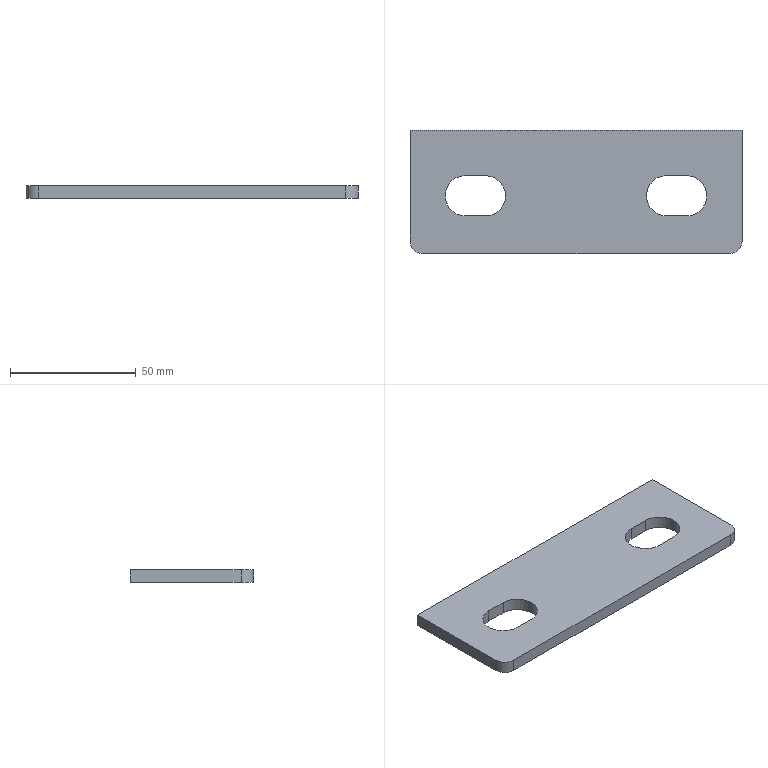Component | SolidWorks | LiftingVerticalBeamAssembly-1_LiftingBasePlate-1 | 1 solid | 18 faces | box 132 x 49 x 5 mm | volume 28996 mm3 | plane 10 | cylinder 8 | commonest cylinder face diameters 16 x6 10 x2 | material Plain Carbon Steel
STEP:
#1=CARTESIAN_POINT('',(73.673,-0.254,79.428));
#2=VERTEX_POINT('',#1);
#3=CARTESIAN_POINT('',(73.358,0.06098,79.428));
#4=VERTEX_POINT('',#3);
#5=CARTESIAN_POINT('',(73.358,-0.254,79.428));
#6=DIRECTION('',(0.,0.,1.));
#7=DIRECTION('',(-1.,0.,0.));
#8=AXIS2_PLACEMENT_3D('',#5,#6,#7);
#9=CIRCLE('',#8,0.315);
#10=EDGE_CURVE('',#2,#4,#9,.T.);
#11=ORIENTED_EDGE('',*,*,#10,.F.);
#12=CARTESIAN_POINT('',(73.673,-0.254,79.625));
#13=VERTEX_POINT('',#12);
#14=CARTESIAN_POINT('',(73.673,-0.254,79.428));
#15=DIRECTION('',(0.,0.,1.));
#16=VECTOR('',#15,39.37);
#17=LINE('',#14,#16);
#18=EDGE_CURVE('',#2,#13,#17,.T.);
#19=ORIENTED_EDGE('',*,*,#18,.T.);
#20=CARTESIAN_POINT('',(73.358,0.06098,79.625));
#21=VERTEX_POINT('',#20);
#22=CARTESIAN_POINT('',(73.358,-0.254,79.625));
#23=DIRECTION('',(0.,0.,1.));
#24=DIRECTION('',(-1.,0.,0.));
#25=AXIS2_PLACEMENT_3D('',#22,#23,#24);
#26=CIRCLE('',#25,0.315);
#27=EDGE_CURVE('',#13,#21,#26,.T.);
#28=ORIENTED_EDGE('',*,*,#27,.T.);
#29=CARTESIAN_POINT('',(73.358,0.06098,79.428));
#30=DIRECTION('',(0.,0.,1.));
#31=VECTOR('',#30,39.37);
#32=LINE('',#29,#31);
#33=EDGE_CURVE('',#4,#21,#32,.T.);
#34=ORIENTED_EDGE('',*,*,#33,.F.);
#35=EDGE_LOOP('',(#11,#19,#28,#34));
#36=FACE_OUTER_BOUND('',#35,.T.);
#37=CARTESIAN_POINT('',(73.358,-0.254,79.428));
#38=DIRECTION('',(0.,0.,1.));
#39=DIRECTION('',(1.,0.,0.));
#40=AXIS2_PLACEMENT_3D('',#37,#38,#39);
#41=CYLINDRICAL_SURFACE('',#40,0.315);
#42=ADVANCED_FACE('',(#36),#41,.F.);
#43=CARTESIAN_POINT('',(70.523,-0.254,79.428));
#44=VERTEX_POINT('',#43);
#45=CARTESIAN_POINT('',(70.208,0.06098,79.428));
#46=VERTEX_POINT('',#45);
#47=CARTESIAN_POINT('',(70.208,-0.254,79.428));
#48=DIRECTION('',(0.,0.,1.));
#49=DIRECTION('',(1.,0.,0.));
#50=AXIS2_PLACEMENT_3D('',#47,#48,#49);
#51=CIRCLE('',#50,0.315);
#52=EDGE_CURVE('',#44,#46,#51,.T.);
#53=ORIENTED_EDGE('',*,*,#52,.F.);
#54=CARTESIAN_POINT('',(70.523,-0.254,79.625));
#55=VERTEX_POINT('',#54);
#56=CARTESIAN_POINT('',(70.523,-0.254,79.428));
#57=DIRECTION('',(0.,0.,1.));
#58=VECTOR('',#57,39.37);
#59=LINE('',#56,#58);
#60=EDGE_CURVE('',#44,#55,#59,.T.);
#61=ORIENTED_EDGE('',*,*,#60,.T.);
#62=CARTESIAN_POINT('',(70.208,0.06098,79.625));
#63=VERTEX_POINT('',#62);
#64=CARTESIAN_POINT('',(70.208,-0.254,79.625));
#65=DIRECTION('',(0.,0.,1.));
#66=DIRECTION('',(1.,0.,0.));
#67=AXIS2_PLACEMENT_3D('',#64,#65,#66);
#68=CIRCLE('',#67,0.315);
#69=EDGE_CURVE('',#55,#63,#68,.T.);
#70=ORIENTED_EDGE('',*,*,#69,.T.);
#71=CARTESIAN_POINT('',(70.208,0.06098,79.428));
#72=DIRECTION('',(0.,0.,1.));
#73=VECTOR('',#72,39.37);
#74=LINE('',#71,#73);
#75=EDGE_CURVE('',#46,#63,#74,.T.);
#76=ORIENTED_EDGE('',*,*,#75,.F.);
#77=EDGE_LOOP('',(#53,#61,#70,#76));
#78=FACE_OUTER_BOUND('',#77,.T.);
#79=CARTESIAN_POINT('',(70.208,-0.254,79.428));
#80=DIRECTION('',(0.,0.,1.));
#81=DIRECTION('',(1.,0.,0.));
#82=AXIS2_PLACEMENT_3D('',#79,#80,#81);
#83=CYLINDRICAL_SURFACE('',#82,0.315);
#84=ADVANCED_FACE('',(#78),#83,.F.);
#85=CARTESIAN_POINT('',(69.027,0.7696,79.428));
#86=VERTEX_POINT('',#85);
#87=CARTESIAN_POINT('',(69.027,-0.9626,79.428));
#88=VERTEX_POINT('',#87);
#89=CARTESIAN_POINT('',(69.027,0.7696,79.428));
#90=DIRECTION('',(0.,-1.,0.));
#91=VECTOR('',#90,39.37);
#92=LINE('',#89,#91);
#93=EDGE_CURVE('',#86,#88,#92,.T.);
#94=ORIENTED_EDGE('',*,*,#93,.T.);
#95=CARTESIAN_POINT('',(69.027,-0.9626,79.625));
#96=VERTEX_POINT('',#95);
#97=CARTESIAN_POINT('',(69.027,-0.9626,79.428));
#98=DIRECTION('',(0.,0.,1.));
#99=VECTOR('',#98,39.37);
#100=LINE('',#97,#99);
#101=EDGE_CURVE('',#88,#96,#100,.T.);
#102=ORIENTED_EDGE('',*,*,#101,.T.);
#103=CARTESIAN_POINT('',(69.027,0.7696,79.625));
#104=VERTEX_POINT('',#103);
#105=CARTESIAN_POINT('',(69.027,0.7696,79.625));
#106=DIRECTION('',(0.,-1.,0.));
#107=VECTOR('',#106,39.37);
#108=LINE('',#105,#107);
#109=EDGE_CURVE('',#104,#96,#108,.T.);
#110=ORIENTED_EDGE('',*,*,#109,.F.);
#111=CARTESIAN_POINT('',(69.027,0.7696,79.428));
#112=DIRECTION('',(0.,0.,1.));
#113=VECTOR('',#112,39.37);
#114=LINE('',#111,#113);
#115=EDGE_CURVE('',#86,#104,#114,.T.);
#116=ORIENTED_EDGE('',*,*,#115,.F.);
#117=EDGE_LOOP('',(#94,#102,#110,#116));
#118=FACE_OUTER_BOUND('',#117,.T.);
#119=CARTESIAN_POINT('',(69.027,0.7696,79.428));
#120=DIRECTION('',(-1.,-0.,0.));
#121=DIRECTION('',(0.,-1.,0.));
#122=AXIS2_PLACEMENT_3D('',#119,#120,#121);
#123=PLANE('',#122);
#124=ADVANCED_FACE('',(#118),#123,.T.);
#125=CARTESIAN_POINT('',(74.224,0.7696,79.625));
#126=VERTEX_POINT('',#125);
#127=CARTESIAN_POINT('',(69.027,0.7696,79.625));
#128=DIRECTION('',(-1.,0.,0.));
#129=VECTOR('',#128,39.37);
#130=LINE('',#127,#129);
#131=EDGE_CURVE('',#126,#104,#130,.T.);
#132=ORIENTED_EDGE('',*,*,#131,.F.);
#133=CARTESIAN_POINT('',(74.224,0.7696,79.428));
#134=VERTEX_POINT('',#133);
#135=CARTESIAN_POINT('',(74.224,0.7696,79.428));
#136=DIRECTION('',(0.,0.,1.));
#137=VECTOR('',#136,39.37);
#138=LINE('',#135,#137);
#139=EDGE_CURVE('',#134,#126,#138,.T.);
#140=ORIENTED_EDGE('',*,*,#139,.F.);
#141=CARTESIAN_POINT('',(69.027,0.7696,79.428));
#142=DIRECTION('',(-1.,0.,0.));
#143=VECTOR('',#142,39.37);
#144=LINE('',#141,#143);
#145=EDGE_CURVE('',#134,#86,#144,.T.);
#146=ORIENTED_EDGE('',*,*,#145,.T.);
#147=ORIENTED_EDGE('',*,*,#115,.T.);
#148=EDGE_LOOP('',(#132,#140,#146,#147));
#149=FACE_OUTER_BOUND('',#148,.T.);
#150=CARTESIAN_POINT('',(69.027,0.7696,79.428));
#151=DIRECTION('',(0.,1.,0.));
#152=DIRECTION('',(0.,0.,1.));
#153=AXIS2_PLACEMENT_3D('',#150,#151,#152);
#154=PLANE('',#153);
#155=ADVANCED_FACE('',(#149),#154,.T.);
#156=CARTESIAN_POINT('',(74.224,-0.9626,79.625));
#157=VERTEX_POINT('',#156);
#158=CARTESIAN_POINT('',(74.224,0.7696,79.625));
#159=DIRECTION('',(0.,1.,0.));
#160=VECTOR('',#159,39.37);
#161=LINE('',#158,#160);
#162=EDGE_CURVE('',#157,#126,#161,.T.);
#163=ORIENTED_EDGE('',*,*,#162,.F.);
#164=CARTESIAN_POINT('',(74.224,-0.9626,79.428));
#165=VERTEX_POINT('',#164);
#166=CARTESIAN_POINT('',(74.224,-0.9626,79.428));
#167=DIRECTION('',(0.,0.,-1.));
#168=VECTOR('',#167,39.37);
#169=LINE('',#166,#168);
#170=EDGE_CURVE('',#157,#165,#169,.T.);
#171=ORIENTED_EDGE('',*,*,#170,.T.);
#172=CARTESIAN_POINT('',(74.224,0.7696,79.428));
#173=DIRECTION('',(0.,1.,0.));
#174=VECTOR('',#173,39.37);
#175=LINE('',#172,#174);
#176=EDGE_CURVE('',#165,#134,#175,.T.);
#177=ORIENTED_EDGE('',*,*,#176,.T.);
#178=ORIENTED_EDGE('',*,*,#139,.T.);
#179=EDGE_LOOP('',(#163,#171,#177,#178));
#180=FACE_OUTER_BOUND('',#179,.T.);
#181=CARTESIAN_POINT('',(74.224,0.7696,79.428));
#182=DIRECTION('',(1.,0.,0.));
#183=DIRECTION('',(0.,0.,-1.));
#184=AXIS2_PLACEMENT_3D('',#181,#182,#183);
#185=PLANE('',#184);
#186=ADVANCED_FACE('',(#180),#185,.T.);
#187=CARTESIAN_POINT('',(69.224,-1.159,79.428));
#188=VERTEX_POINT('',#187);
#189=CARTESIAN_POINT('',(74.027,-1.159,79.428));
#190=VERTEX_POINT('',#189);
#191=CARTESIAN_POINT('',(69.027,-1.159,79.428));
#192=DIRECTION('',(1.,0.,0.));
#193=VECTOR('',#192,39.37);
#194=LINE('',#191,#193);
#195=EDGE_CURVE('',#188,#190,#194,.T.);
#196=ORIENTED_EDGE('',*,*,#195,.T.);
#197=CARTESIAN_POINT('',(74.027,-1.159,79.625));
#198=VERTEX_POINT('',#197);
#199=CARTESIAN_POINT('',(74.027,-1.159,79.428));
#200=DIRECTION('',(0.,0.,1.));
#201=VECTOR('',#200,39.37);
#202=LINE('',#199,#201);
#203=EDGE_CURVE('',#190,#198,#202,.T.);
#204=ORIENTED_EDGE('',*,*,#203,.T.);
#205=CARTESIAN_POINT('',(69.224,-1.159,79.625));
#206=VERTEX_POINT('',#205);
#207=CARTESIAN_POINT('',(69.027,-1.159,79.625));
#208=DIRECTION('',(1.,0.,0.));
#209=VECTOR('',#208,39.37);
#210=LINE('',#207,#209);
#211=EDGE_CURVE('',#206,#198,#210,.T.);
#212=ORIENTED_EDGE('',*,*,#211,.F.);
#213=CARTESIAN_POINT('',(69.224,-1.159,79.428));
#214=DIRECTION('',(0.,0.,-1.));
#215=VECTOR('',#214,39.37);
#216=LINE('',#213,#215);
#217=EDGE_CURVE('',#206,#188,#216,.T.);
#218=ORIENTED_EDGE('',*,*,#217,.T.);
#219=EDGE_LOOP('',(#196,#204,#212,#218));
#220=FACE_OUTER_BOUND('',#219,.T.);
#221=CARTESIAN_POINT('',(69.027,-1.159,79.428));
#222=DIRECTION('',(0.,-1.,0.));
#223=DIRECTION('',(0.,0.,-1.));
#224=AXIS2_PLACEMENT_3D('',#221,#222,#223);
#225=PLANE('',#224);
#226=ADVANCED_FACE('',(#220),#225,.T.);
#227=CARTESIAN_POINT('',(73.043,-0.5689,79.428));
#228=VERTEX_POINT('',#227);
#229=CARTESIAN_POINT('',(73.358,-0.5689,79.428));
#230=VERTEX_POINT('',#229);
#231=CARTESIAN_POINT('',(73.358,-0.5689,79.428));
#232=DIRECTION('',(1.,0.,0.));
#233=VECTOR('',#232,39.37);
#234=LINE('',#231,#233);
#235=EDGE_CURVE('',#228,#230,#234,.T.);
#236=ORIENTED_EDGE('',*,*,#235,.T.);
#237=CARTESIAN_POINT('',(73.358,-0.254,79.428));
#238=DIRECTION('',(0.,0.,1.));
#239=DIRECTION('',(-1.,0.,0.));
#240=AXIS2_PLACEMENT_3D('',#237,#238,#239);
#241=CIRCLE('',#240,0.315);
#242=EDGE_CURVE('',#230,#2,#241,.T.);
#243=ORIENTED_EDGE('',*,*,#242,.T.);
#244=ORIENTED_EDGE('',*,*,#10,.T.);
#245=CARTESIAN_POINT('',(73.043,0.06098,79.428));
#246=VERTEX_POINT('',#245);
#247=CARTESIAN_POINT('',(73.358,0.06098,79.428));
#248=DIRECTION('',(-1.,0.,0.));
#249=VECTOR('',#248,39.37);
#250=LINE('',#247,#249);
#251=EDGE_CURVE('',#4,#246,#250,.T.);
#252=ORIENTED_EDGE('',*,*,#251,.T.);
#253=CARTESIAN_POINT('',(73.043,-0.254,79.428));
#254=DIRECTION('',(0.,0.,1.));
#255=DIRECTION('',(-1.,0.,0.));
#256=AXIS2_PLACEMENT_3D('',#253,#254,#255);
#257=CIRCLE('',#256,0.315);
#258=EDGE_CURVE('',#246,#228,#257,.T.);
#259=ORIENTED_EDGE('',*,*,#258,.T.);
#260=EDGE_LOOP('',(#236,#243,#244,#252,#259));
#261=FACE_BOUND('',#260,.T.);
#262=CARTESIAN_POINT('',(69.893,0.06098,79.428));
#263=VERTEX_POINT('',#262);
#264=CARTESIAN_POINT('',(69.893,0.06098,79.428));
#265=DIRECTION('',(-1.,0.,0.));
#266=VECTOR('',#265,39.37);
#267=LINE('',#264,#266);
#268=EDGE_CURVE('',#46,#263,#267,.T.);
#269=ORIENTED_EDGE('',*,*,#268,.T.);
#270=CARTESIAN_POINT('',(69.893,-0.5689,79.428));
#271=VERTEX_POINT('',#270);
#272=CARTESIAN_POINT('',(69.893,-0.254,79.428));
#273=DIRECTION('',(0.,0.,1.));
#274=DIRECTION('',(1.,0.,0.));
#275=AXIS2_PLACEMENT_3D('',#272,#273,#274);
#276=CIRCLE('',#275,0.315);
#277=EDGE_CURVE('',#263,#271,#276,.T.);
#278=ORIENTED_EDGE('',*,*,#277,.T.);
#279=CARTESIAN_POINT('',(70.208,-0.5689,79.428));
#280=VERTEX_POINT('',#279);
#281=CARTESIAN_POINT('',(69.893,-0.5689,79.428));
#282=DIRECTION('',(1.,0.,0.));
#283=VECTOR('',#282,39.37);
#284=LINE('',#281,#283);
#285=EDGE_CURVE('',#271,#280,#284,.T.);
#286=ORIENTED_EDGE('',*,*,#285,.T.);
#287=CARTESIAN_POINT('',(70.208,-0.254,79.428));
#288=DIRECTION('',(0.,0.,1.));
#289=DIRECTION('',(1.,0.,0.));
#290=AXIS2_PLACEMENT_3D('',#287,#288,#289);
#291=CIRCLE('',#290,0.315);
#292=EDGE_CURVE('',#280,#44,#291,.T.);
#293=ORIENTED_EDGE('',*,*,#292,.T.);
#294=ORIENTED_EDGE('',*,*,#52,.T.);
#295=EDGE_LOOP('',(#269,#278,#286,#293,#294));
#296=FACE_BOUND('',#295,.T.);
#297=ORIENTED_EDGE('',*,*,#176,.F.);
#298=CARTESIAN_POINT('',(74.027,-0.9626,79.428));
#299=DIRECTION('',(0.,0.,-1.));
#300=DIRECTION('',(1.,0.,0.));
#301=AXIS2_PLACEMENT_3D('',#298,#299,#300);
#302=CIRCLE('',#301,0.1969);
#303=EDGE_CURVE('',#165,#190,#302,.T.);
#304=ORIENTED_EDGE('',*,*,#303,.T.);
#305=ORIENTED_EDGE('',*,*,#195,.F.);
#306=CARTESIAN_POINT('',(69.224,-0.9626,79.428));
#307=DIRECTION('',(0.,0.,-1.));
#308=DIRECTION('',(1.,0.,0.));
#309=AXIS2_PLACEMENT_3D('',#306,#307,#308);
#310=CIRCLE('',#309,0.1969);
#311=EDGE_CURVE('',#188,#88,#310,.T.);
#312=ORIENTED_EDGE('',*,*,#311,.T.);
#313=ORIENTED_EDGE('',*,*,#93,.F.);
#314=ORIENTED_EDGE('',*,*,#145,.F.);
#315=EDGE_LOOP('',(#297,#304,#305,#312,#313,#314));
#316=FACE_OUTER_BOUND('',#315,.T.);
#317=CARTESIAN_POINT('',(69.027,-1.159,79.428));
#318=DIRECTION('',(0.,0.,1.));
#319=DIRECTION('',(1.,0.,0.));
#320=AXIS2_PLACEMENT_3D('',#317,#318,#319);
#321=PLANE('',#320);
#322=ADVANCED_FACE('',(#261,#296,#316),#321,.F.);
#323=CARTESIAN_POINT('',(73.358,-0.5689,79.625));
#324=VERTEX_POINT('',#323);
#325=CARTESIAN_POINT('',(73.358,-0.254,79.625));
#326=DIRECTION('',(0.,0.,1.));
#327=DIRECTION('',(-1.,0.,0.));
#328=AXIS2_PLACEMENT_3D('',#325,#326,#327);
#329=CIRCLE('',#328,0.315);
#330=EDGE_CURVE('',#324,#13,#329,.T.);
#331=ORIENTED_EDGE('',*,*,#330,.F.);
#332=CARTESIAN_POINT('',(73.043,-0.5689,79.625));
#333=VERTEX_POINT('',#332);
#334=CARTESIAN_POINT('',(73.358,-0.5689,79.625));
#335=DIRECTION('',(1.,0.,0.));
#336=VECTOR('',#335,39.37);
#337=LINE('',#334,#336);
#338=EDGE_CURVE('',#333,#324,#337,.T.);
#339=ORIENTED_EDGE('',*,*,#338,.F.);
#340=CARTESIAN_POINT('',(73.043,0.06098,79.625));
#341=VERTEX_POINT('',#340);
#342=CARTESIAN_POINT('',(73.043,-0.254,79.625));
#343=DIRECTION('',(0.,0.,1.));
#344=DIRECTION('',(-1.,0.,0.));
#345=AXIS2_PLACEMENT_3D('',#342,#343,#344);
#346=CIRCLE('',#345,0.315);
#347=EDGE_CURVE('',#341,#333,#346,.T.);
#348=ORIENTED_EDGE('',*,*,#347,.F.);
#349=CARTESIAN_POINT('',(73.358,0.06098,79.625));
#350=DIRECTION('',(-1.,0.,0.));
#351=VECTOR('',#350,39.37);
#352=LINE('',#349,#351);
#353=EDGE_CURVE('',#21,#341,#352,.T.);
#354=ORIENTED_EDGE('',*,*,#353,.F.);
#355=ORIENTED_EDGE('',*,*,#27,.F.);
#356=EDGE_LOOP('',(#331,#339,#348,#354,#355));
#357=FACE_BOUND('',#356,.T.);
#358=CARTESIAN_POINT('',(69.893,0.06098,79.625));
#359=VERTEX_POINT('',#358);
#360=CARTESIAN_POINT('',(69.893,-0.5689,79.625));
#361=VERTEX_POINT('',#360);
#362=CARTESIAN_POINT('',(69.893,-0.254,79.625));
#363=DIRECTION('',(0.,0.,1.));
#364=DIRECTION('',(1.,0.,0.));
#365=AXIS2_PLACEMENT_3D('',#362,#363,#364);
#366=CIRCLE('',#365,0.315);
#367=EDGE_CURVE('',#359,#361,#366,.T.);
#368=ORIENTED_EDGE('',*,*,#367,.F.);
#369=CARTESIAN_POINT('',(69.893,0.06098,79.625));
#370=DIRECTION('',(-1.,0.,0.));
#371=VECTOR('',#370,39.37);
#372=LINE('',#369,#371);
#373=EDGE_CURVE('',#63,#359,#372,.T.);
#374=ORIENTED_EDGE('',*,*,#373,.F.);
#375=ORIENTED_EDGE('',*,*,#69,.F.);
#376=CARTESIAN_POINT('',(70.208,-0.5689,79.625));
#377=VERTEX_POINT('',#376);
#378=CARTESIAN_POINT('',(70.208,-0.254,79.625));
#379=DIRECTION('',(0.,0.,1.));
#380=DIRECTION('',(1.,0.,0.));
#381=AXIS2_PLACEMENT_3D('',#378,#379,#380);
#382=CIRCLE('',#381,0.315);
#383=EDGE_CURVE('',#377,#55,#382,.T.);
#384=ORIENTED_EDGE('',*,*,#383,.F.);
#385=CARTESIAN_POINT('',(69.893,-0.5689,79.625));
#386=DIRECTION('',(1.,0.,0.));
#387=VECTOR('',#386,39.37);
#388=LINE('',#385,#387);
#389=EDGE_CURVE('',#361,#377,#388,.T.);
#390=ORIENTED_EDGE('',*,*,#389,.F.);
#391=EDGE_LOOP('',(#368,#374,#375,#384,#390));
#392=FACE_BOUND('',#391,.T.);
#393=ORIENTED_EDGE('',*,*,#211,.T.);
#394=CARTESIAN_POINT('',(74.027,-0.9626,79.625));
#395=DIRECTION('',(0.,0.,1.));
#396=DIRECTION('',(1.,0.,0.));
#397=AXIS2_PLACEMENT_3D('',#394,#395,#396);
#398=CIRCLE('',#397,0.1969);
#399=EDGE_CURVE('',#198,#157,#398,.T.);
#400=ORIENTED_EDGE('',*,*,#399,.T.);
#401=ORIENTED_EDGE('',*,*,#162,.T.);
#402=ORIENTED_EDGE('',*,*,#131,.T.);
#403=ORIENTED_EDGE('',*,*,#109,.T.);
#404=CARTESIAN_POINT('',(69.224,-0.9626,79.625));
#405=DIRECTION('',(0.,0.,1.));
#406=DIRECTION('',(1.,0.,0.));
#407=AXIS2_PLACEMENT_3D('',#404,#405,#406);
#408=CIRCLE('',#407,0.1969);
#409=EDGE_CURVE('',#96,#206,#408,.T.);
#410=ORIENTED_EDGE('',*,*,#409,.T.);
#411=EDGE_LOOP('',(#393,#400,#401,#402,#403,#410));
#412=FACE_OUTER_BOUND('',#411,.T.);
#413=CARTESIAN_POINT('',(69.027,-1.159,79.625));
#414=DIRECTION('',(0.,0.,1.));
#415=DIRECTION('',(1.,0.,0.));
#416=AXIS2_PLACEMENT_3D('',#413,#414,#415);
#417=PLANE('',#416);
#418=ADVANCED_FACE('',(#357,#392,#412),#417,.T.);
#419=ORIENTED_EDGE('',*,*,#303,.F.);
#420=ORIENTED_EDGE('',*,*,#170,.F.);
#421=ORIENTED_EDGE('',*,*,#399,.F.);
#422=ORIENTED_EDGE('',*,*,#203,.F.);
#423=EDGE_LOOP('',(#419,#420,#421,#422));
#424=FACE_OUTER_BOUND('',#423,.T.);
#425=CARTESIAN_POINT('',(74.027,-0.9626,79.428));
#426=DIRECTION('',(0.,0.,1.));
#427=DIRECTION('',(1.,0.,0.));
#428=AXIS2_PLACEMENT_3D('',#425,#426,#427);
#429=CYLINDRICAL_SURFACE('',#428,0.1969);
#430=ADVANCED_FACE('',(#424),#429,.T.);
#431=ORIENTED_EDGE('',*,*,#311,.F.);
#432=ORIENTED_EDGE('',*,*,#217,.F.);
#433=ORIENTED_EDGE('',*,*,#409,.F.);
#434=ORIENTED_EDGE('',*,*,#101,.F.);
#435=EDGE_LOOP('',(#431,#432,#433,#434));
#436=FACE_OUTER_BOUND('',#435,.T.);
#437=CARTESIAN_POINT('',(69.224,-0.9626,79.428));
#438=DIRECTION('',(0.,0.,1.));
#439=DIRECTION('',(1.,0.,0.));
#440=AXIS2_PLACEMENT_3D('',#437,#438,#439);
#441=CYLINDRICAL_SURFACE('',#440,0.1969);
#442=ADVANCED_FACE('',(#436),#441,.T.);
#443=ORIENTED_EDGE('',*,*,#367,.T.);
#444=CARTESIAN_POINT('',(69.893,-0.5689,79.428));
#445=DIRECTION('',(0.,0.,1.));
#446=VECTOR('',#445,39.37);
#447=LINE('',#444,#446);
#448=EDGE_CURVE('',#271,#361,#447,.T.);
#449=ORIENTED_EDGE('',*,*,#448,.F.);
#450=ORIENTED_EDGE('',*,*,#277,.F.);
#451=CARTESIAN_POINT('',(69.893,0.06098,79.428));
#452=DIRECTION('',(0.,0.,1.));
#453=VECTOR('',#452,39.37);
#454=LINE('',#451,#453);
#455=EDGE_CURVE('',#263,#359,#454,.T.);
#456=ORIENTED_EDGE('',*,*,#455,.T.);
#457=EDGE_LOOP('',(#443,#449,#450,#456));
#458=FACE_OUTER_BOUND('',#457,.T.);
#459=CARTESIAN_POINT('',(69.893,-0.254,79.428));
#460=DIRECTION('',(0.,0.,1.));
#461=DIRECTION('',(1.,0.,0.));
#462=AXIS2_PLACEMENT_3D('',#459,#460,#461);
#463=CYLINDRICAL_SURFACE('',#462,0.315);
#464=ADVANCED_FACE('',(#458),#463,.F.);
#465=ORIENTED_EDGE('',*,*,#373,.T.);
#466=ORIENTED_EDGE('',*,*,#455,.F.);
#467=ORIENTED_EDGE('',*,*,#268,.F.);
#468=ORIENTED_EDGE('',*,*,#75,.T.);
#469=EDGE_LOOP('',(#465,#466,#467,#468));
#470=FACE_OUTER_BOUND('',#469,.T.);
#471=CARTESIAN_POINT('',(69.893,0.06098,79.428));
#472=DIRECTION('',(0.,1.,0.));
#473=DIRECTION('',(0.,0.,1.));
#474=AXIS2_PLACEMENT_3D('',#471,#472,#473);
#475=PLANE('',#474);
#476=ADVANCED_FACE('',(#470),#475,.F.);
#477=ORIENTED_EDGE('',*,*,#60,.F.);
#478=ORIENTED_EDGE('',*,*,#292,.F.);
#479=CARTESIAN_POINT('',(70.208,-0.5689,79.428));
#480=DIRECTION('',(0.,0.,1.));
#481=VECTOR('',#480,39.37);
#482=LINE('',#479,#481);
#483=EDGE_CURVE('',#280,#377,#482,.T.);
#484=ORIENTED_EDGE('',*,*,#483,.T.);
#485=ORIENTED_EDGE('',*,*,#383,.T.);
#486=EDGE_LOOP('',(#477,#478,#484,#485));
#487=FACE_OUTER_BOUND('',#486,.T.);
#488=CARTESIAN_POINT('',(70.208,-0.254,79.428));
#489=DIRECTION('',(0.,0.,1.));
#490=DIRECTION('',(1.,0.,0.));
#491=AXIS2_PLACEMENT_3D('',#488,#489,#490);
#492=CYLINDRICAL_SURFACE('',#491,0.315);
#493=ADVANCED_FACE('',(#487),#492,.F.);
#494=ORIENTED_EDGE('',*,*,#389,.T.);
#495=ORIENTED_EDGE('',*,*,#483,.F.);
#496=ORIENTED_EDGE('',*,*,#285,.F.);
#497=ORIENTED_EDGE('',*,*,#448,.T.);
#498=EDGE_LOOP('',(#494,#495,#496,#497));
#499=FACE_OUTER_BOUND('',#498,.T.);
#500=CARTESIAN_POINT('',(69.893,-0.5689,79.428));
#501=DIRECTION('',(0.,-1.,0.));
#502=DIRECTION('',(0.,0.,-1.));
#503=AXIS2_PLACEMENT_3D('',#500,#501,#502);
#504=PLANE('',#503);
#505=ADVANCED_FACE('',(#499),#504,.F.);
#506=ORIENTED_EDGE('',*,*,#18,.F.);
#507=ORIENTED_EDGE('',*,*,#242,.F.);
#508=CARTESIAN_POINT('',(73.358,-0.5689,79.428));
#509=DIRECTION('',(0.,0.,1.));
#510=VECTOR('',#509,39.37);
#511=LINE('',#508,#510);
#512=EDGE_CURVE('',#230,#324,#511,.T.);
#513=ORIENTED_EDGE('',*,*,#512,.T.);
#514=ORIENTED_EDGE('',*,*,#330,.T.);
#515=EDGE_LOOP('',(#506,#507,#513,#514));
#516=FACE_OUTER_BOUND('',#515,.T.);
#517=CARTESIAN_POINT('',(73.358,-0.254,79.428));
#518=DIRECTION('',(0.,0.,1.));
#519=DIRECTION('',(1.,0.,0.));
#520=AXIS2_PLACEMENT_3D('',#517,#518,#519);
#521=CYLINDRICAL_SURFACE('',#520,0.315);
#522=ADVANCED_FACE('',(#516),#521,.F.);
#523=ORIENTED_EDGE('',*,*,#338,.T.);
#524=ORIENTED_EDGE('',*,*,#512,.F.);
#525=ORIENTED_EDGE('',*,*,#235,.F.);
#526=CARTESIAN_POINT('',(73.043,-0.5689,79.428));
#527=DIRECTION('',(0.,0.,1.));
#528=VECTOR('',#527,39.37);
#529=LINE('',#526,#528);
#530=EDGE_CURVE('',#228,#333,#529,.T.);
#531=ORIENTED_EDGE('',*,*,#530,.T.);
#532=EDGE_LOOP('',(#523,#524,#525,#531));
#533=FACE_OUTER_BOUND('',#532,.T.);
#534=CARTESIAN_POINT('',(73.358,-0.5689,79.428));
#535=DIRECTION('',(0.,-1.,0.));
#536=DIRECTION('',(1.,0.,0.));
#537=AXIS2_PLACEMENT_3D('',#534,#535,#536);
#538=PLANE('',#537);
#539=ADVANCED_FACE('',(#533),#538,.F.);
#540=ORIENTED_EDGE('',*,*,#347,.T.);
#541=ORIENTED_EDGE('',*,*,#530,.F.);
#542=ORIENTED_EDGE('',*,*,#258,.F.);
#543=CARTESIAN_POINT('',(73.043,0.06098,79.428));
#544=DIRECTION('',(0.,0.,1.));
#545=VECTOR('',#544,39.37);
#546=LINE('',#543,#545);
#547=EDGE_CURVE('',#246,#341,#546,.T.);
#548=ORIENTED_EDGE('',*,*,#547,.T.);
#549=EDGE_LOOP('',(#540,#541,#542,#548));
#550=FACE_OUTER_BOUND('',#549,.T.);
#551=CARTESIAN_POINT('',(73.043,-0.254,79.428));
#552=DIRECTION('',(0.,0.,1.));
#553=DIRECTION('',(1.,0.,0.));
#554=AXIS2_PLACEMENT_3D('',#551,#552,#553);
#555=CYLINDRICAL_SURFACE('',#554,0.315);
#556=ADVANCED_FACE('',(#550),#555,.F.);
#557=ORIENTED_EDGE('',*,*,#353,.T.);
#558=ORIENTED_EDGE('',*,*,#547,.F.);
#559=ORIENTED_EDGE('',*,*,#251,.F.);
#560=ORIENTED_EDGE('',*,*,#33,.T.);
#561=EDGE_LOOP('',(#557,#558,#559,#560));
#562=FACE_OUTER_BOUND('',#561,.T.);
#563=CARTESIAN_POINT('',(73.358,0.06098,79.428));
#564=DIRECTION('',(0.,1.,0.));
#565=DIRECTION('',(0.,0.,1.));
#566=AXIS2_PLACEMENT_3D('',#563,#564,#565);
#567=PLANE('',#566);
#568=ADVANCED_FACE('',(#562),#567,.F.);
#569=CLOSED_SHELL('',(#42,#84,#124,#155,#186,#226,#322,#418,#430,#442,#464,#476,#493,#505,#522,#539,#556,#568));
#570=MANIFOLD_SOLID_BREP('',#569);
#571=CARTESIAN_POINT('',(0.,0.,0.));
#572=DIRECTION('',(0.,0.,1.));
#573=DIRECTION('',(1.,0.,0.));
#574=AXIS2_PLACEMENT_3D('',#571,#572,#573);
#575=(LENGTH_UNIT()NAMED_UNIT(*)SI_UNIT($,.METRE.));
#576=LENGTH_MEASURE_WITH_UNIT(LENGTH_MEASURE(0.0254),#575);
#577=DIMENSIONAL_EXPONENTS(1.,0.,0.,0.,0.,0.,0.);
#578=(CONVERSION_BASED_UNIT('',#576)LENGTH_UNIT()NAMED_UNIT(#577));
#579=UNCERTAINTY_MEASURE_WITH_UNIT(LENGTH_MEASURE(0.00001),#578,'','');
#580=(NAMED_UNIT(*)PLANE_ANGLE_UNIT()SI_UNIT($,.RADIAN.));
#581=(NAMED_UNIT(*)SI_UNIT($,.STERADIAN.)SOLID_ANGLE_UNIT());
#582=(GEOMETRIC_REPRESENTATION_CONTEXT(3)GLOBAL_UNCERTAINTY_ASSIGNED_CONTEXT((#579))GLOBAL_UNIT_ASSIGNED_CONTEXT((#578,#580,#581))REPRESENTATION_CONTEXT('',''));
#583=ADVANCED_BREP_SHAPE_REPRESENTATION('',(#570,#574),#582);
#584=COLOUR_RGB('',0.7922,0.8196,0.9333);
#585=FILL_AREA_STYLE_COLOUR('',#584);
#586=FILL_AREA_STYLE('',(#585));
#587=SURFACE_STYLE_FILL_AREA(#586);
#588=SURFACE_SIDE_STYLE('',(#587));
#589=SURFACE_STYLE_USAGE(.BOTH.,#588);
#590=PRESENTATION_STYLE_ASSIGNMENT((#589));
#591=STYLED_ITEM('',(#590),#570);
#592=PRESENTATION_LAYER_ASSIGNMENT('','',(#591));
#593=(LENGTH_UNIT()NAMED_UNIT(*)SI_UNIT($,.METRE.));
#594=LENGTH_MEASURE_WITH_UNIT(LENGTH_MEASURE(0.0254),#593);
#595=DIMENSIONAL_EXPONENTS(1.,0.,0.,0.,0.,0.,0.);
#596=(CONVERSION_BASED_UNIT('',#594)LENGTH_UNIT()NAMED_UNIT(#595));
#597=UNCERTAINTY_MEASURE_WITH_UNIT(LENGTH_MEASURE(0.00001),#596,'','');
#598=(NAMED_UNIT(*)PLANE_ANGLE_UNIT()SI_UNIT($,.RADIAN.));
#599=(NAMED_UNIT(*)SI_UNIT($,.STERADIAN.)SOLID_ANGLE_UNIT());
#600=(GEOMETRIC_REPRESENTATION_CONTEXT(3)GLOBAL_UNCERTAINTY_ASSIGNED_CONTEXT((#597))GLOBAL_UNIT_ASSIGNED_CONTEXT((#596,#598,#599))REPRESENTATION_CONTEXT('',''));
#601=MECHANICAL_DESIGN_GEOMETRIC_PRESENTATION_REPRESENTATION('',(#591),#600);